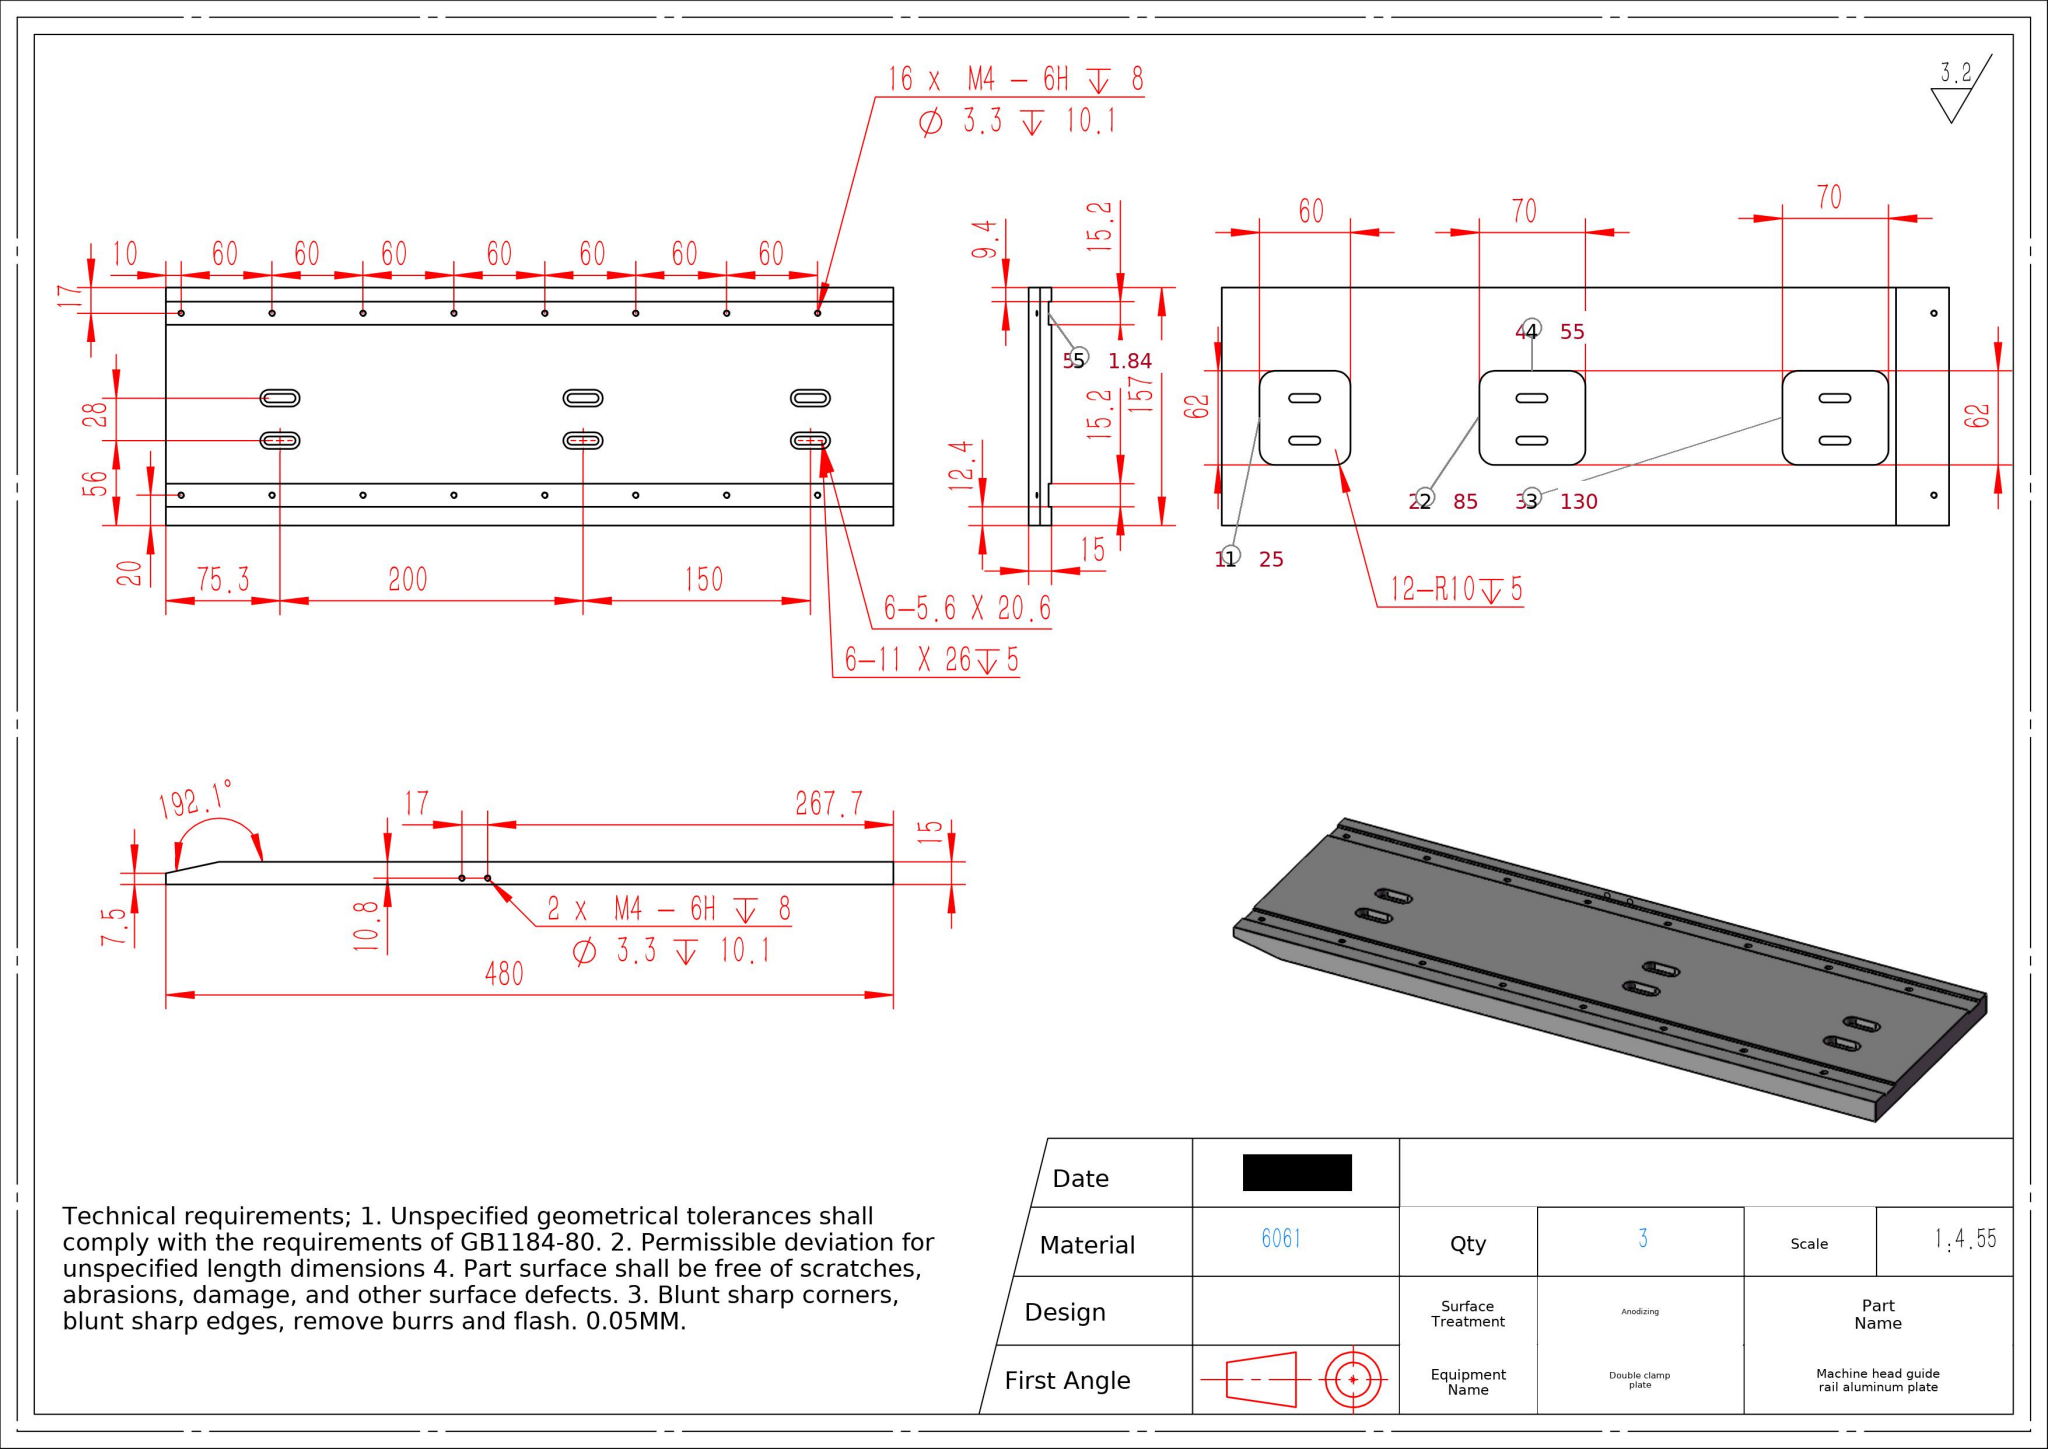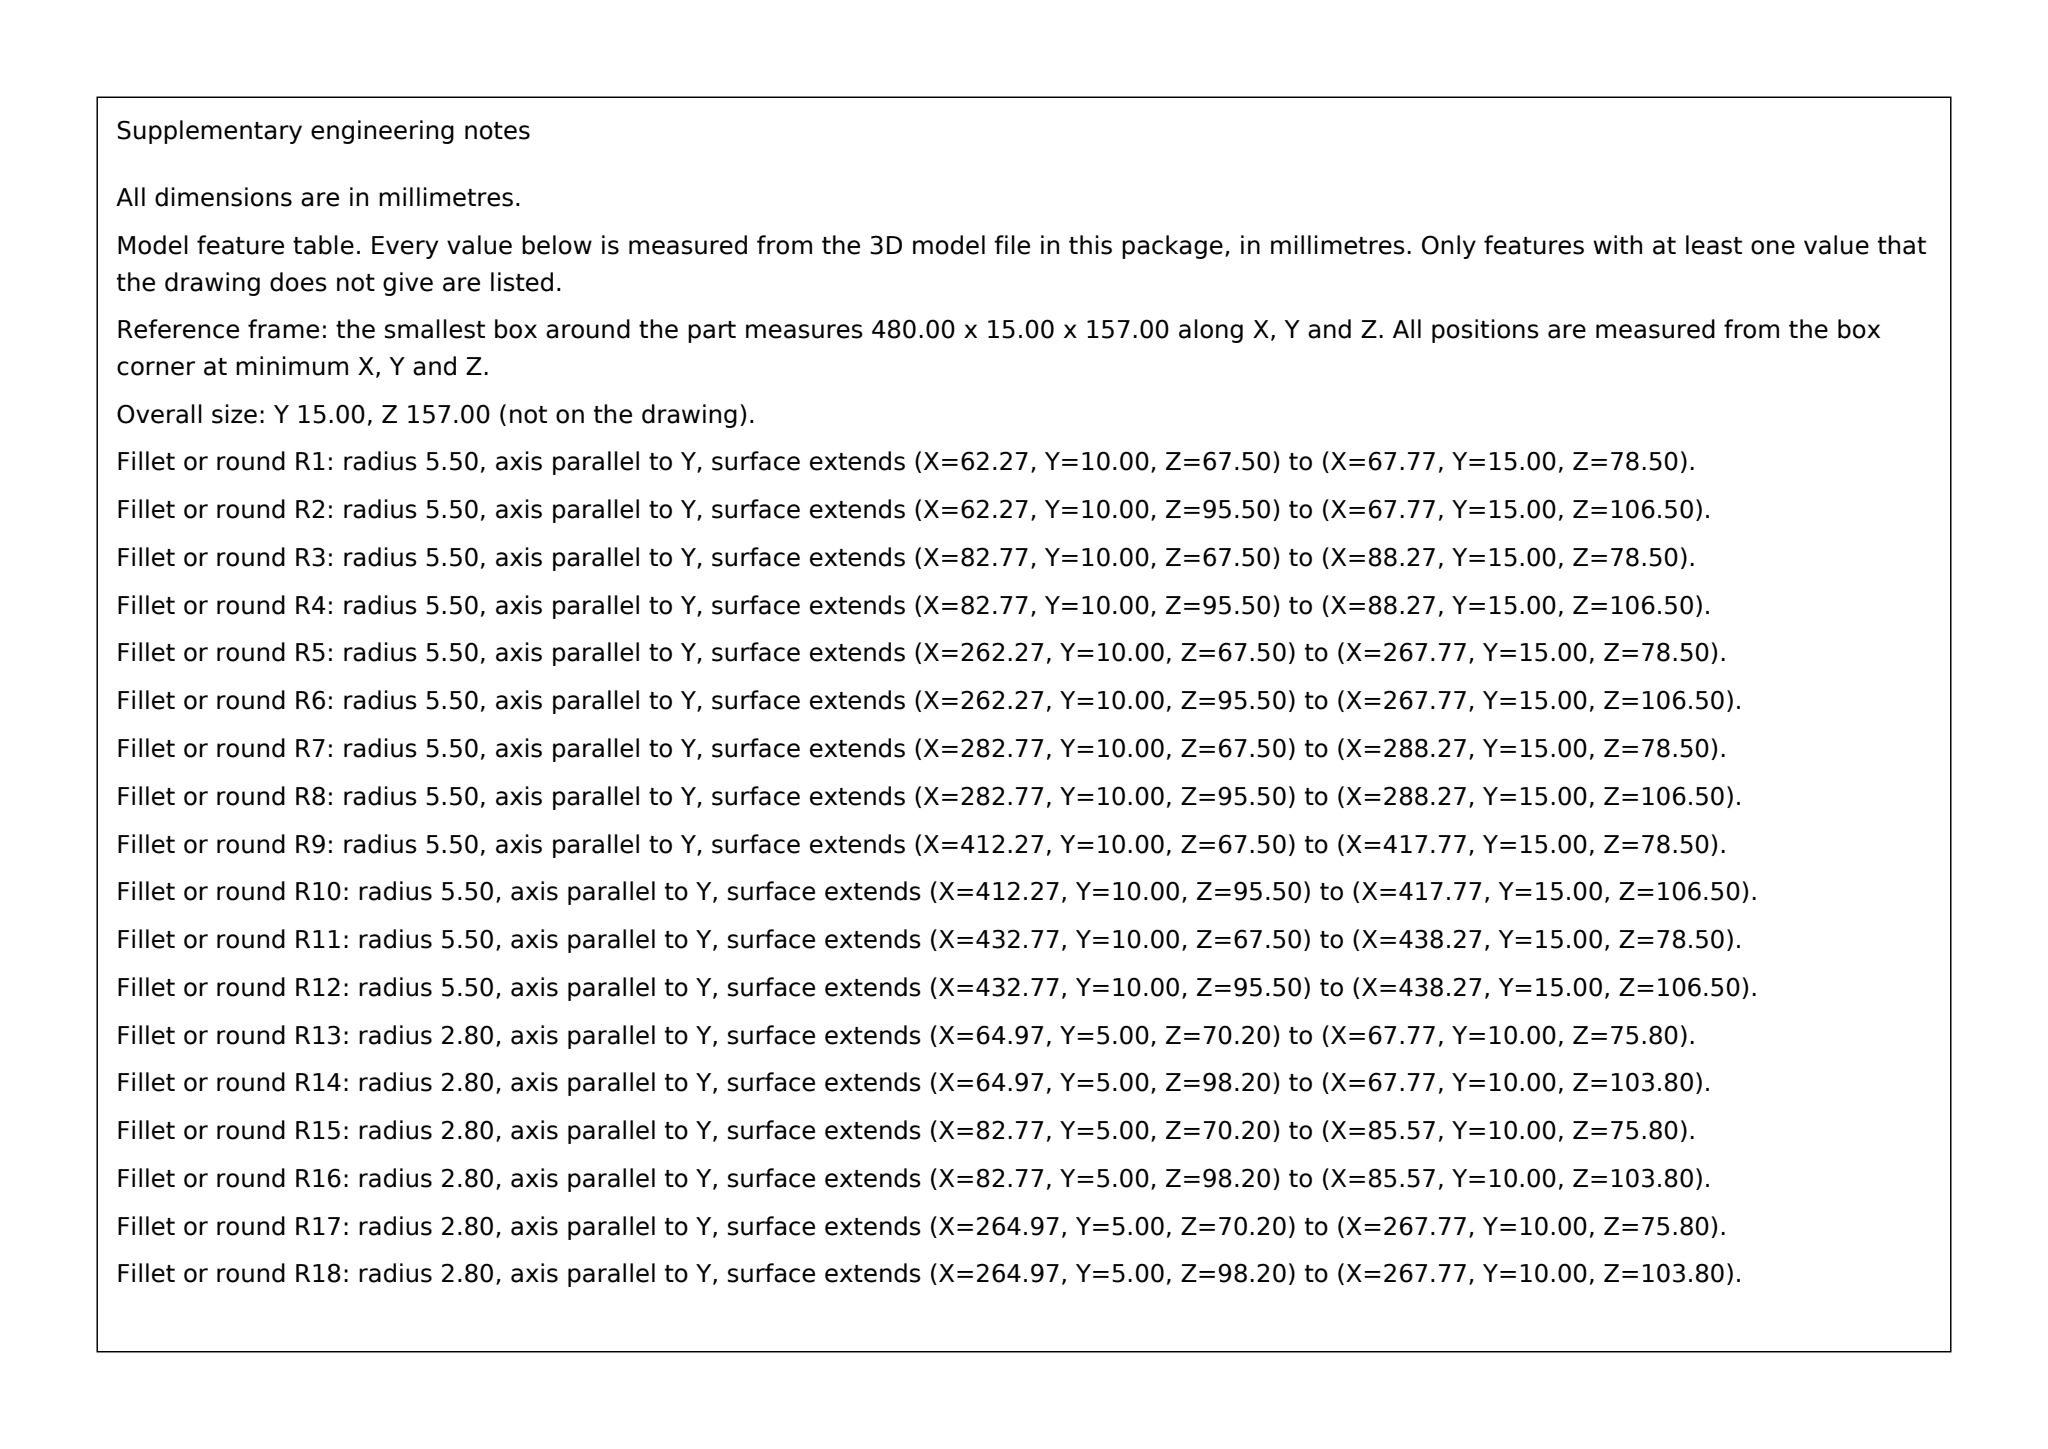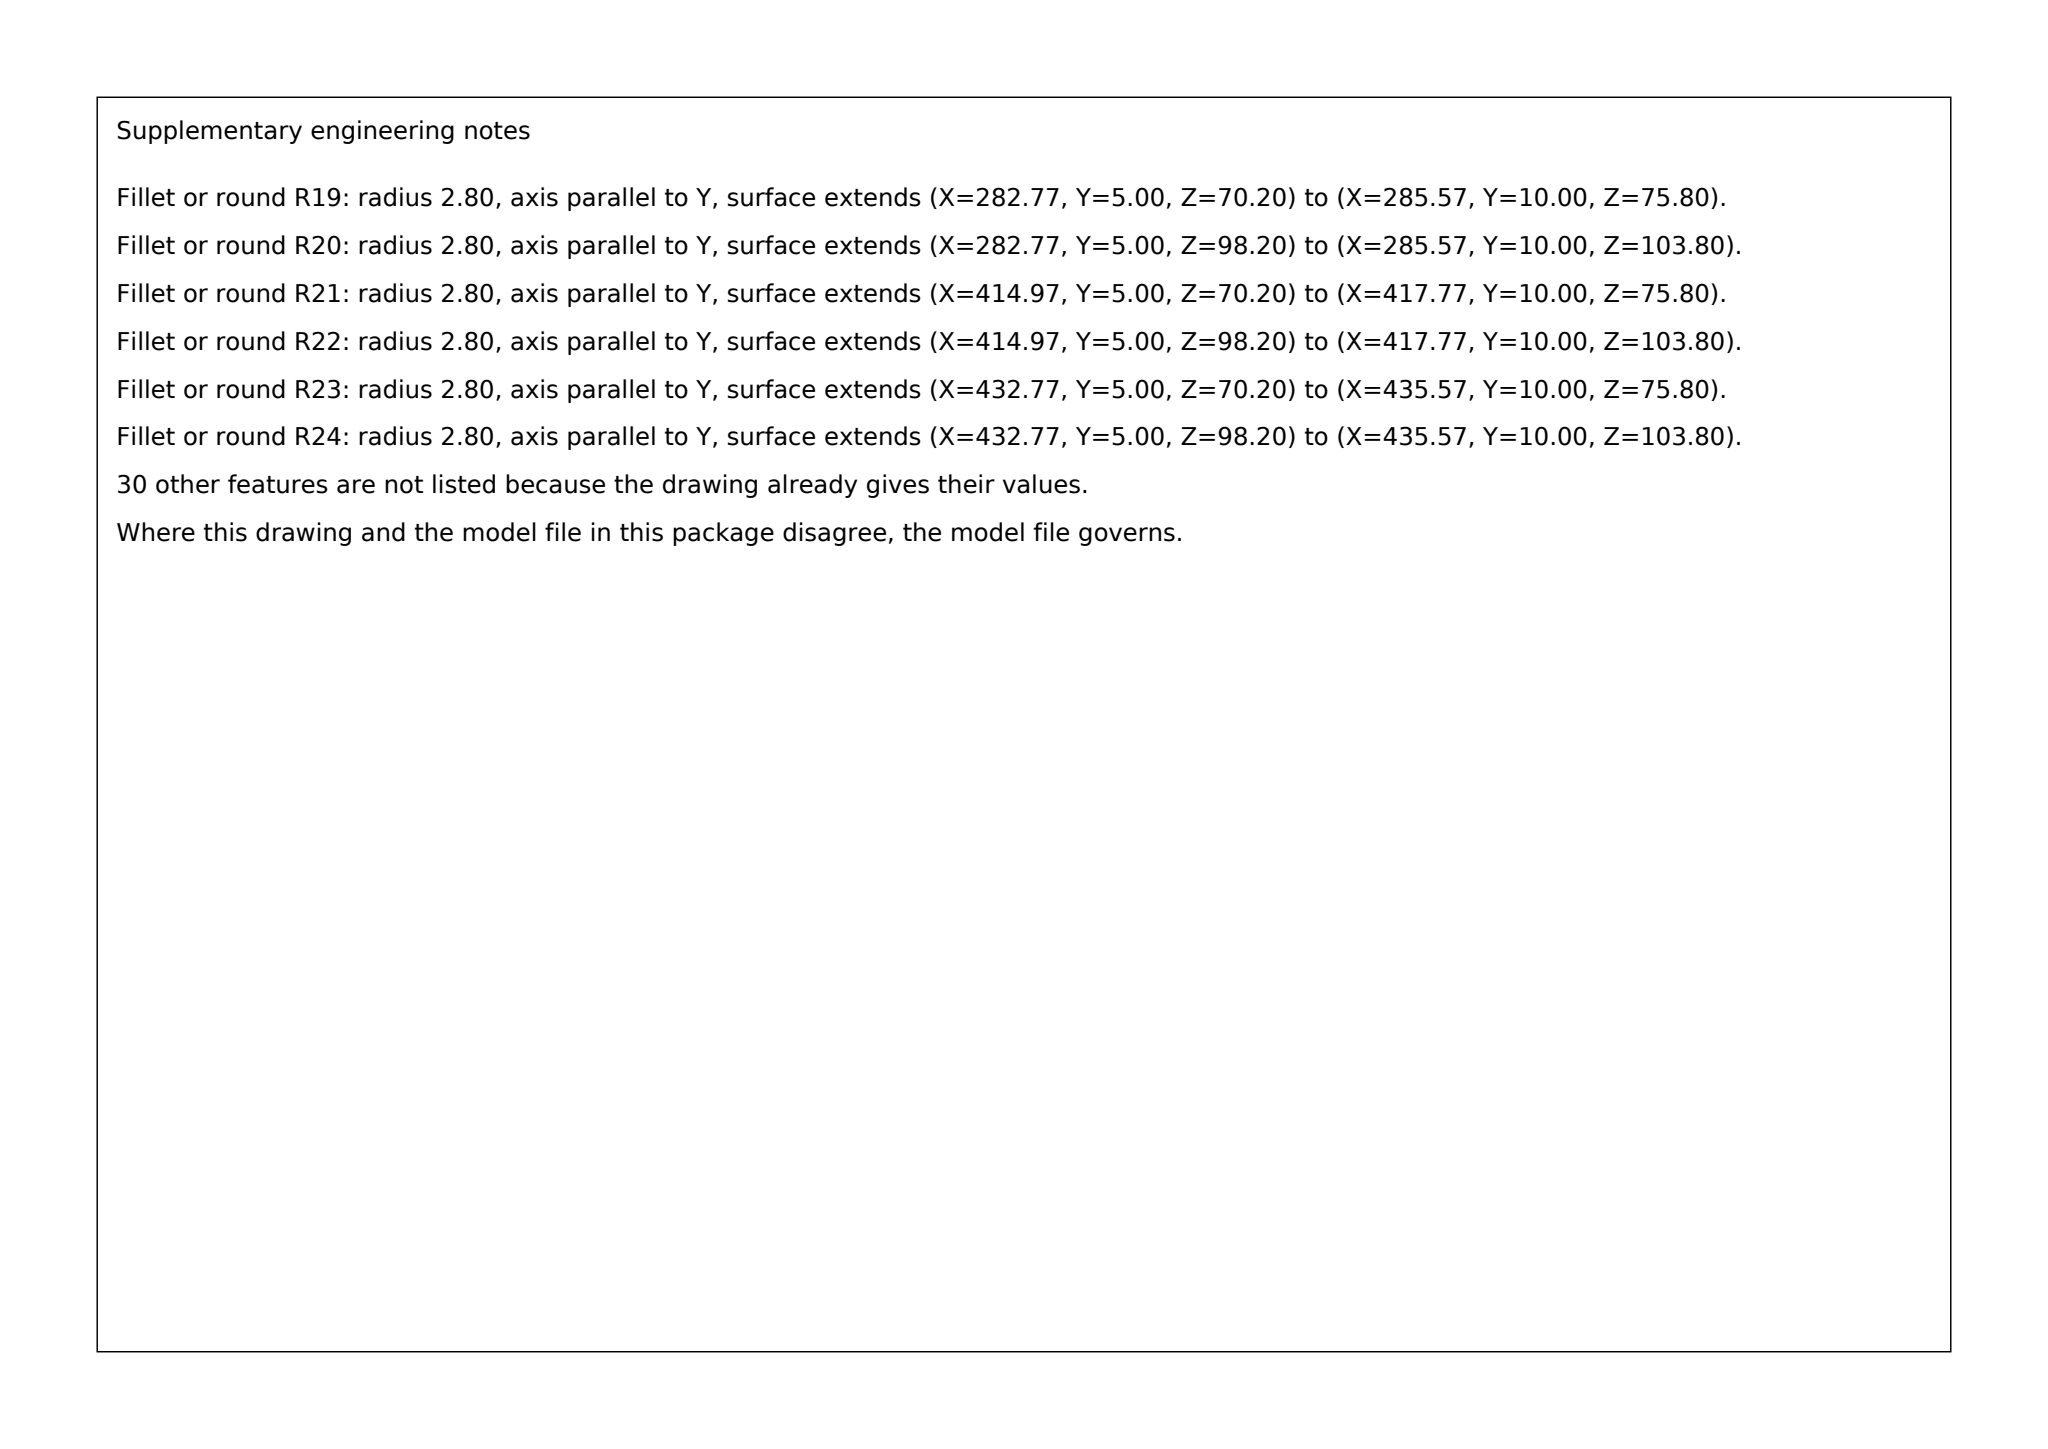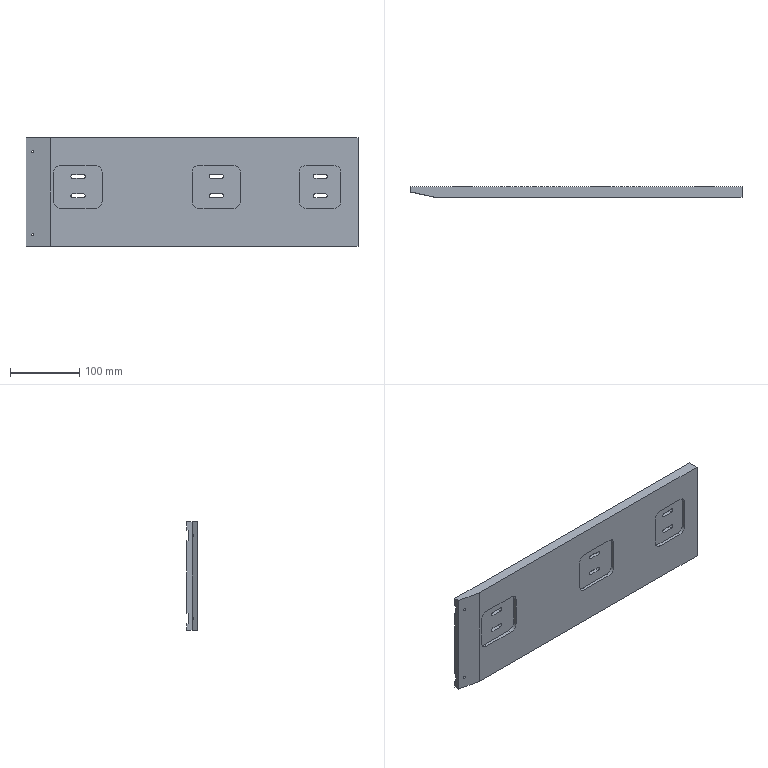Part | SolidWorks | mm | material 6061 | 1 solid | 162 faces | box 480 x 15 x 157 mm | volume 1009617 mm3 | cylinder 72 | plane 62 | cone 28 | commonest cylinder face diameters 3.3 x36 11 x12 5.6 x12 20 x12
build123d program:
from build123d import *

# Parameters (mm, degrees)
BOSS_EXTRUDE1_DEPTH   = 157
SKETCH2_W             = 15.2
SKETCH2_H             = 1.84
CUT_EXTRUDE1_DEPTH    = 489.608
SKETCH3_W             = 15.2
SKETCH3_H             = 1.84
CUT_EXTRUDE2_DEPTH    = 489.608
SKETCH4_W             = 70
SKETCH4_H             = 62
CUT_EXTRUDE3_DEPTH    = 5
SKETCH9_W             = 70
SKETCH9_H             = 62
CUT_EXTRUDE8_DEPTH    = 5
CUT_EXTRUDE9_DEPTH    = 5
CUT_EXTRUDE10_DEPTH   = 275.099
CUT_EXTRUDE11_DEPTH   = 5
CUT_EXTRUDE12_DEPTH   = 275.099
SKETCH14_W            = 60
SKETCH14_H            = 62
CUT_EXTRUDE13_DEPTH   = 5
M4_TAPPED_HOLE1_D     = 3.3
M4_TAPPED_HOLE1_DEPTH = 10.1
M4_TAPPED_HOLE2_D     = 3.3
M4_TAPPED_HOLE2_DEPTH = 10.1
M4_TAPPED_HOLE2_TIP   = 0.9914
M4_TAPPED_HOLE3_D     = 3.3
FILLET1_R             = 10
LPATTERN1_COUNT       = 2
LPATTERN1_PITCH       = 200
LPATTERN2_COUNT       = 2
LPATTERN2_PITCH       = 150


with BuildPart() as part:
    # Sketch1 → Boss-Extrude1 (new body)
    with BuildSketch(Plane.XY.offset(70)):
        Polygon((-220.267, 20.23), (-185.267, 12.73), (259.733, 12.73), (259.733, 27.73), (-220.267, 27.73), align=None)
    extrude(amount=-BOSS_EXTRUDE1_DEPTH)

    # Sketch2 → Cut-Extrude1 (cut, through all)
    with BuildSketch(Plane(origin=(259.733, 0, 0), x_dir=(0, 0, -1), z_dir=(1, 0, 0))):
        with Locations((-50, 26.81)):
            Rectangle(SKETCH2_W, SKETCH2_H)
    extrude(amount=-CUT_EXTRUDE1_DEPTH, mode=Mode.SUBTRACT)

    # Sketch3 → Cut-Extrude2 (cut, through all)
    with BuildSketch(Plane(origin=(259.733, 0, 0), x_dir=(0, 0, -1), z_dir=(1, 0, 0))):
        with Locations((70, 26.81)):
            Rectangle(SKETCH3_W, SKETCH3_H)
    extrude(amount=-CUT_EXTRUDE2_DEPTH, mode=Mode.SUBTRACT)

    # Sketch4 → Cut-Extrude3 (cut)
    with BuildSketch(Plane.XZ.offset(-12.73)):
        with Locations((-145.267, -1)):
            Rectangle(SKETCH4_W, SKETCH4_H)
    extrude(amount=-CUT_EXTRUDE3_DEPTH, mode=Mode.SUBTRACT)

    # Sketch9 → Cut-Extrude8 (cut)
    with BuildSketch(Plane.XZ.offset(-12.73)):
        with Locations((54.733, -1)):
            Rectangle(SKETCH9_W, SKETCH9_H)
    extrude(amount=-CUT_EXTRUDE8_DEPTH, mode=Mode.SUBTRACT)

    # Sketch10 → Cut-Extrude9 (cut)
    with BuildSketch(Plane(origin=(0, 27.73, 0), x_dir=(-1, 0, 0), z_dir=(0, 1, 0))):
        with BuildLine():
            Line((-62.503, -8.5), (-47.503, -8.5))
            ThreePointArc((-47.503, -8.5), (-42.003, -14), (-47.503, -19.5))
            Line((-47.503, -19.5), (-62.503, -19.5))
            ThreePointArc((-62.503, -19.5), (-68.003, -14), (-62.503, -8.5))
        make_face()
    cut_extrude9 = extrude(amount=-CUT_EXTRUDE9_DEPTH, mode=Mode.SUBTRACT)

    # Sketch11 → Cut-Extrude10 (cut, through all)
    with BuildSketch(Plane.XZ.offset(-17.73)):
        with BuildLine():
            Line((47.503, -11.2), (62.503, -11.2))
            ThreePointArc((62.503, -11.2), (65.303, -14), (62.503, -16.8))
            Line((62.503, -16.8), (47.503, -16.8))
            ThreePointArc((47.503, -16.8), (44.703, -14), (47.503, -11.2))
        make_face()
    cut_extrude10 = extrude(amount=-CUT_EXTRUDE10_DEPTH, mode=Mode.SUBTRACT)

    # Sketch12 → Cut-Extrude11 (cut)
    with BuildSketch(Plane(origin=(0, 27.73, 0), x_dir=(-1, 0, 0), z_dir=(0, 1, 0))):
        with BuildLine():
            Line((-62.503, 19.5), (-47.503, 19.5))
            ThreePointArc((-47.503, 19.5), (-42.003, 14), (-47.503, 8.5))
            Line((-47.503, 8.5), (-62.503, 8.5))
            ThreePointArc((-62.503, 8.5), (-68.003, 14), (-62.503, 19.5))
        make_face()
    cut_extrude11 = extrude(amount=-CUT_EXTRUDE11_DEPTH, mode=Mode.SUBTRACT)

    # Sketch13 → Cut-Extrude12 (cut, through all)
    with BuildSketch(Plane(origin=(0, 22.73, 0), x_dir=(-1, 0, 0), z_dir=(0, 1, 0))):
        with BuildLine():
            Line((-62.503, 16.8), (-47.503, 16.8))
            ThreePointArc((-47.503, 16.8), (-44.703, 14), (-47.503, 11.2))
            Line((-47.503, 11.2), (-62.503, 11.2))
            ThreePointArc((-62.503, 11.2), (-65.303, 14), (-62.503, 16.8))
        make_face()
    cut_extrude12 = extrude(amount=-CUT_EXTRUDE12_DEPTH, mode=Mode.SUBTRACT)

    # Sketch14 → Cut-Extrude13 (cut)
    with BuildSketch(Plane.XZ.offset(-12.73)):
        with Locations((204.733, -1)):
            Rectangle(SKETCH14_W, SKETCH14_H)
    extrude(amount=-CUT_EXTRUDE13_DEPTH, mode=Mode.SUBTRACT)

    # M4 Tapped Hole1
    with Locations(Plane(origin=(0, 0, -87), x_dir=(-1, 0, 0), z_dir=(0, 0, -1))):
        with Locations((8, 23.5), (25, 23.5)):
            Hole(M4_TAPPED_HOLE1_D / 2, depth=M4_TAPPED_HOLE1_DEPTH)

    # M4 Tapped Hole2
    with Locations(Plane(origin=(0, 25.89, 0), x_dir=(1, 0, 0), z_dir=(0, 1, 0))):
        with Locations((-150.267, -50), (-150.267, 70), (-90.267, -50), (-90.267, 70), (-30.267, -50), (-30.267, 70), (29.733, -50), (29.733, 70), (89.733, -50), (89.733, 70), (149.733, -50), (149.733, 70), (209.733, -50), (209.733, 70)):
            Hole(M4_TAPPED_HOLE2_D / 2, depth=M4_TAPPED_HOLE2_DEPTH)
            with Locations((0, 0, -(M4_TAPPED_HOLE2_DEPTH + M4_TAPPED_HOLE2_TIP / 2))):  # 118° drill point
                Cone(0, M4_TAPPED_HOLE2_D / 2, M4_TAPPED_HOLE2_TIP, mode=Mode.SUBTRACT)

    # M4 Tapped Hole3 (through all)
    with Locations(Plane(origin=(0, 25.89, 0), x_dir=(1, 0, 0), z_dir=(0, 1, 0))):
        with Locations((-210.267, -50), (-210.267, 70)):
            Hole(M4_TAPPED_HOLE3_D / 2)

    # Fillet1
    fillet1_edges = [part.edges().sort_by_distance(p)[0] for p in [
        (174.733, 15.23, 30),
        (234.733, 15.23, 30),
        (234.733, 15.23, -32),
        (174.733, 15.23, -32),
        (-110.267, 15.23, 30),
        (-110.267, 15.23, -32),
        (-180.267, 15.23, -32),
        (-180.267, 15.23, 30),
        (19.733, 15.23, 30),
        (89.733, 15.23, 30),
        (89.733, 15.23, -32),
        (19.733, 15.23, -32),
    ]]
    fillet(fillet1_edges, radius=FILLET1_R)

    # LPattern1: Cut-Extrude9, Cut-Extrude10, Cut-Extrude11, Cut-Extrude12 ×2
    with Locations(*[(-i * LPATTERN1_PITCH, 0, 0) for i in range(1, LPATTERN1_COUNT)]):
        add(cut_extrude9, mode=Mode.SUBTRACT)
        add(cut_extrude10, mode=Mode.SUBTRACT)
        add(cut_extrude11, mode=Mode.SUBTRACT)
        add(cut_extrude12, mode=Mode.SUBTRACT)

    # LPattern2: Cut-Extrude9, Cut-Extrude10, Cut-Extrude11, Cut-Extrude12 ×2
    with Locations(*[(i * LPATTERN2_PITCH, 0, 0) for i in range(1, LPATTERN2_COUNT)]):
        add(cut_extrude9, mode=Mode.SUBTRACT)
        add(cut_extrude10, mode=Mode.SUBTRACT)
        add(cut_extrude11, mode=Mode.SUBTRACT)
        add(cut_extrude12, mode=Mode.SUBTRACT)


solid = part.part